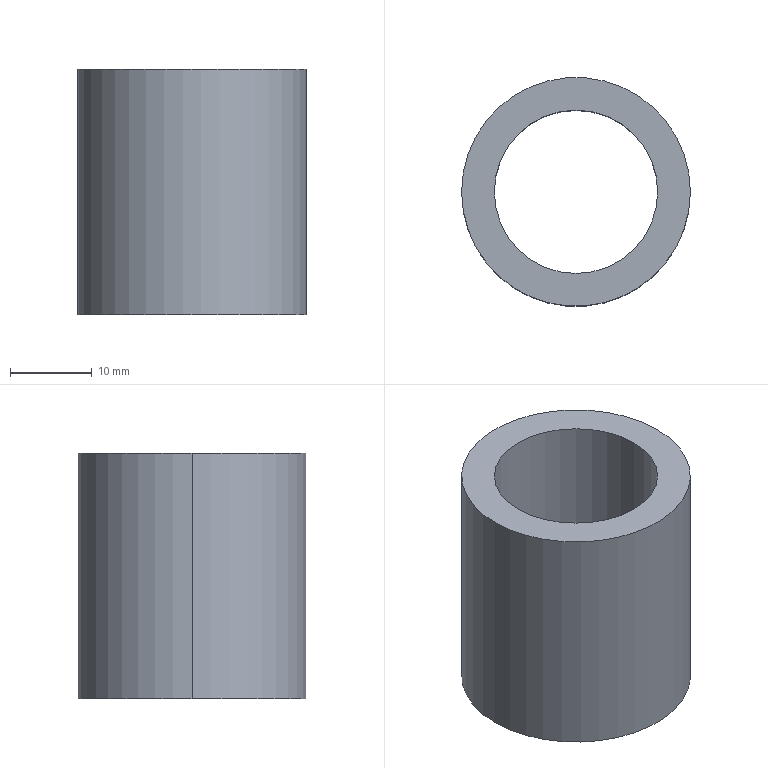Component | SolidWorks | GraphiteCopperSleeve2--1 | 1 solid | 6 faces | box 28 x 28 x 30 mm | volume 9048 mm3 | cylinder 4 | plane 2 | commonest cylinder face diameters 20 x2 28 x2
build123d program:
from build123d import *

# Parameters (mm, degrees)
SKETCH1_R           = 14
SKETCH1_R_2         = 10
BOSS_EXTRUDE1_DEPTH = 30


with BuildPart() as part:
    # Sketch1 → Boss-Extrude1 (new body)
    with BuildSketch(Plane.XY):
        Circle(SKETCH1_R)
        Circle(SKETCH1_R_2, mode=Mode.SUBTRACT)
    extrude(amount=BOSS_EXTRUDE1_DEPTH)


solid = part.part

# Placed as in the assembly
solid = solid.moved(Location((-372.766, -43.543, 885), (0, 0, 0)))
STEP:
#1=CARTESIAN_POINT('',(-15.07,-1.714,36.024));
#2=VERTEX_POINT('',#1);
#3=CARTESIAN_POINT('',(-14.282,-1.714,36.024));
#4=VERTEX_POINT('',#3);
#5=CARTESIAN_POINT('',(-14.676,-1.714,36.024));
#6=DIRECTION('',(0.,-0.,1.));
#7=DIRECTION('',(1.,0.,0.));
#8=AXIS2_PLACEMENT_3D('',#5,#6,#7);
#9=CIRCLE('',#8,0.3937);
#10=EDGE_CURVE('',#2,#4,#9,.T.);
#11=ORIENTED_EDGE('',*,*,#10,.T.);
#12=CARTESIAN_POINT('',(-14.282,-1.714,34.843));
#13=VERTEX_POINT('',#12);
#14=CARTESIAN_POINT('',(-14.282,-1.714,36.024));
#15=DIRECTION('',(-0.,0.,-1.));
#16=VECTOR('',#15,39.37);
#17=LINE('',#14,#16);
#18=EDGE_CURVE('',#4,#13,#17,.T.);
#19=ORIENTED_EDGE('',*,*,#18,.T.);
#20=CARTESIAN_POINT('',(-15.07,-1.714,34.843));
#21=VERTEX_POINT('',#20);
#22=CARTESIAN_POINT('',(-14.676,-1.714,34.843));
#23=DIRECTION('',(0.,-0.,1.));
#24=DIRECTION('',(1.,0.,0.));
#25=AXIS2_PLACEMENT_3D('',#22,#23,#24);
#26=CIRCLE('',#25,0.3937);
#27=EDGE_CURVE('',#21,#13,#26,.T.);
#28=ORIENTED_EDGE('',*,*,#27,.F.);
#29=CARTESIAN_POINT('',(-15.07,-1.714,36.024));
#30=DIRECTION('',(-0.,0.,-1.));
#31=VECTOR('',#30,39.37);
#32=LINE('',#29,#31);
#33=EDGE_CURVE('',#2,#21,#32,.T.);
#34=ORIENTED_EDGE('',*,*,#33,.F.);
#35=EDGE_LOOP('',(#11,#19,#28,#34));
#36=FACE_OUTER_BOUND('',#35,.T.);
#37=CARTESIAN_POINT('',(-14.676,-1.714,36.024));
#38=DIRECTION('',(-0.,0.,-1.));
#39=DIRECTION('',(-1.,-0.,0.));
#40=AXIS2_PLACEMENT_3D('',#37,#38,#39);
#41=CYLINDRICAL_SURFACE('',#40,0.3937);
#42=ADVANCED_FACE('',(#36),#41,.F.);
#43=CARTESIAN_POINT('',(-14.125,-1.714,36.024));
#44=VERTEX_POINT('',#43);
#45=CARTESIAN_POINT('',(-15.227,-1.714,36.024));
#46=VERTEX_POINT('',#45);
#47=CARTESIAN_POINT('',(-14.676,-1.714,36.024));
#48=DIRECTION('',(0.,-0.,1.));
#49=DIRECTION('',(1.,0.,0.));
#50=AXIS2_PLACEMENT_3D('',#47,#48,#49);
#51=CIRCLE('',#50,0.5512);
#52=EDGE_CURVE('',#44,#46,#51,.T.);
#53=ORIENTED_EDGE('',*,*,#52,.F.);
#54=CARTESIAN_POINT('',(-14.125,-1.714,34.843));
#55=VERTEX_POINT('',#54);
#56=CARTESIAN_POINT('',(-14.125,-1.714,36.024));
#57=DIRECTION('',(-0.,0.,-1.));
#58=VECTOR('',#57,39.37);
#59=LINE('',#56,#58);
#60=EDGE_CURVE('',#44,#55,#59,.T.);
#61=ORIENTED_EDGE('',*,*,#60,.T.);
#62=CARTESIAN_POINT('',(-15.227,-1.714,34.843));
#63=VERTEX_POINT('',#62);
#64=CARTESIAN_POINT('',(-14.676,-1.714,34.843));
#65=DIRECTION('',(0.,-0.,1.));
#66=DIRECTION('',(1.,0.,0.));
#67=AXIS2_PLACEMENT_3D('',#64,#65,#66);
#68=CIRCLE('',#67,0.5512);
#69=EDGE_CURVE('',#55,#63,#68,.T.);
#70=ORIENTED_EDGE('',*,*,#69,.T.);
#71=CARTESIAN_POINT('',(-15.227,-1.714,36.024));
#72=DIRECTION('',(-0.,0.,-1.));
#73=VECTOR('',#72,39.37);
#74=LINE('',#71,#73);
#75=EDGE_CURVE('',#46,#63,#74,.T.);
#76=ORIENTED_EDGE('',*,*,#75,.F.);
#77=EDGE_LOOP('',(#53,#61,#70,#76));
#78=FACE_OUTER_BOUND('',#77,.T.);
#79=CARTESIAN_POINT('',(-14.676,-1.714,36.024));
#80=DIRECTION('',(-0.,0.,-1.));
#81=DIRECTION('',(-1.,-0.,0.));
#82=AXIS2_PLACEMENT_3D('',#79,#80,#81);
#83=CYLINDRICAL_SURFACE('',#82,0.5512);
#84=ADVANCED_FACE('',(#78),#83,.T.);
#85=CARTESIAN_POINT('',(-14.676,-1.714,36.024));
#86=DIRECTION('',(0.,-0.,1.));
#87=DIRECTION('',(1.,0.,0.));
#88=AXIS2_PLACEMENT_3D('',#85,#86,#87);
#89=CIRCLE('',#88,0.5512);
#90=EDGE_CURVE('',#46,#44,#89,.T.);
#91=ORIENTED_EDGE('',*,*,#90,.T.);
#92=ORIENTED_EDGE('',*,*,#52,.T.);
#93=EDGE_LOOP('',(#91,#92));
#94=FACE_OUTER_BOUND('',#93,.T.);
#95=ORIENTED_EDGE('',*,*,#10,.F.);
#96=CARTESIAN_POINT('',(-14.676,-1.714,36.024));
#97=DIRECTION('',(0.,-0.,1.));
#98=DIRECTION('',(1.,0.,0.));
#99=AXIS2_PLACEMENT_3D('',#96,#97,#98);
#100=CIRCLE('',#99,0.3937);
#101=EDGE_CURVE('',#4,#2,#100,.T.);
#102=ORIENTED_EDGE('',*,*,#101,.F.);
#103=EDGE_LOOP('',(#95,#102));
#104=FACE_BOUND('',#103,.T.);
#105=CARTESIAN_POINT('',(-14.676,-1.714,36.024));
#106=DIRECTION('',(0.,-0.,1.));
#107=DIRECTION('',(1.,0.,-0.));
#108=AXIS2_PLACEMENT_3D('',#105,#106,#107);
#109=PLANE('',#108);
#110=ADVANCED_FACE('',(#94,#104),#109,.T.);
#111=CARTESIAN_POINT('',(-14.676,-1.714,34.843));
#112=DIRECTION('',(0.,-0.,1.));
#113=DIRECTION('',(1.,0.,0.));
#114=AXIS2_PLACEMENT_3D('',#111,#112,#113);
#115=CIRCLE('',#114,0.5512);
#116=EDGE_CURVE('',#63,#55,#115,.T.);
#117=ORIENTED_EDGE('',*,*,#116,.F.);
#118=ORIENTED_EDGE('',*,*,#69,.F.);
#119=EDGE_LOOP('',(#117,#118));
#120=FACE_OUTER_BOUND('',#119,.T.);
#121=ORIENTED_EDGE('',*,*,#27,.T.);
#122=CARTESIAN_POINT('',(-14.676,-1.714,34.843));
#123=DIRECTION('',(0.,-0.,1.));
#124=DIRECTION('',(1.,0.,0.));
#125=AXIS2_PLACEMENT_3D('',#122,#123,#124);
#126=CIRCLE('',#125,0.3937);
#127=EDGE_CURVE('',#13,#21,#126,.T.);
#128=ORIENTED_EDGE('',*,*,#127,.T.);
#129=EDGE_LOOP('',(#121,#128));
#130=FACE_BOUND('',#129,.T.);
#131=CARTESIAN_POINT('',(-14.676,-1.714,34.843));
#132=DIRECTION('',(0.,-0.,1.));
#133=DIRECTION('',(1.,0.,-0.));
#134=AXIS2_PLACEMENT_3D('',#131,#132,#133);
#135=PLANE('',#134);
#136=ADVANCED_FACE('',(#120,#130),#135,.F.);
#137=ORIENTED_EDGE('',*,*,#60,.F.);
#138=ORIENTED_EDGE('',*,*,#90,.F.);
#139=ORIENTED_EDGE('',*,*,#75,.T.);
#140=ORIENTED_EDGE('',*,*,#116,.T.);
#141=EDGE_LOOP('',(#137,#138,#139,#140));
#142=FACE_OUTER_BOUND('',#141,.T.);
#143=CARTESIAN_POINT('',(-14.676,-1.714,36.024));
#144=DIRECTION('',(-0.,0.,-1.));
#145=DIRECTION('',(-1.,-0.,0.));
#146=AXIS2_PLACEMENT_3D('',#143,#144,#145);
#147=CYLINDRICAL_SURFACE('',#146,0.5512);
#148=ADVANCED_FACE('',(#142),#147,.T.);
#149=ORIENTED_EDGE('',*,*,#18,.F.);
#150=ORIENTED_EDGE('',*,*,#101,.T.);
#151=ORIENTED_EDGE('',*,*,#33,.T.);
#152=ORIENTED_EDGE('',*,*,#127,.F.);
#153=EDGE_LOOP('',(#149,#150,#151,#152));
#154=FACE_OUTER_BOUND('',#153,.T.);
#155=CARTESIAN_POINT('',(-14.676,-1.714,36.024));
#156=DIRECTION('',(-0.,0.,-1.));
#157=DIRECTION('',(-1.,-0.,0.));
#158=AXIS2_PLACEMENT_3D('',#155,#156,#157);
#159=CYLINDRICAL_SURFACE('',#158,0.3937);
#160=ADVANCED_FACE('',(#154),#159,.F.);
#161=CLOSED_SHELL('',(#42,#84,#110,#136,#148,#160));
#162=MANIFOLD_SOLID_BREP('',#161);
#163=CARTESIAN_POINT('',(0.,0.,0.));
#164=DIRECTION('',(0.,0.,1.));
#165=DIRECTION('',(1.,0.,0.));
#166=AXIS2_PLACEMENT_3D('',#163,#164,#165);
#167=(LENGTH_UNIT()NAMED_UNIT(*)SI_UNIT($,.METRE.));
#168=LENGTH_MEASURE_WITH_UNIT(LENGTH_MEASURE(0.0254),#167);
#169=DIMENSIONAL_EXPONENTS(1.,0.,0.,0.,0.,0.,0.);
#170=(CONVERSION_BASED_UNIT('',#168)LENGTH_UNIT()NAMED_UNIT(#169));
#171=UNCERTAINTY_MEASURE_WITH_UNIT(LENGTH_MEASURE(0.00001),#170,'','');
#172=(NAMED_UNIT(*)PLANE_ANGLE_UNIT()SI_UNIT($,.RADIAN.));
#173=(NAMED_UNIT(*)SI_UNIT($,.STERADIAN.)SOLID_ANGLE_UNIT());
#174=(GEOMETRIC_REPRESENTATION_CONTEXT(3)GLOBAL_UNCERTAINTY_ASSIGNED_CONTEXT((#171))GLOBAL_UNIT_ASSIGNED_CONTEXT((#170,#172,#173))REPRESENTATION_CONTEXT('',''));
#175=ADVANCED_BREP_SHAPE_REPRESENTATION('',(#162,#166),#174);
#176=COLOUR_RGB('',0.7922,0.8196,0.9333);
#177=FILL_AREA_STYLE_COLOUR('',#176);
#178=FILL_AREA_STYLE('',(#177));
#179=SURFACE_STYLE_FILL_AREA(#178);
#180=SURFACE_SIDE_STYLE('',(#179));
#181=SURFACE_STYLE_USAGE(.BOTH.,#180);
#182=PRESENTATION_STYLE_ASSIGNMENT((#181));
#183=STYLED_ITEM('',(#182),#162);
#184=PRESENTATION_LAYER_ASSIGNMENT('','',(#183));
#185=(LENGTH_UNIT()NAMED_UNIT(*)SI_UNIT($,.METRE.));
#186=LENGTH_MEASURE_WITH_UNIT(LENGTH_MEASURE(0.0254),#185);
#187=DIMENSIONAL_EXPONENTS(1.,0.,0.,0.,0.,0.,0.);
#188=(CONVERSION_BASED_UNIT('',#186)LENGTH_UNIT()NAMED_UNIT(#187));
#189=UNCERTAINTY_MEASURE_WITH_UNIT(LENGTH_MEASURE(0.00001),#188,'','');
#190=(NAMED_UNIT(*)PLANE_ANGLE_UNIT()SI_UNIT($,.RADIAN.));
#191=(NAMED_UNIT(*)SI_UNIT($,.STERADIAN.)SOLID_ANGLE_UNIT());
#192=(GEOMETRIC_REPRESENTATION_CONTEXT(3)GLOBAL_UNCERTAINTY_ASSIGNED_CONTEXT((#189))GLOBAL_UNIT_ASSIGNED_CONTEXT((#188,#190,#191))REPRESENTATION_CONTEXT('',''));
#193=MECHANICAL_DESIGN_GEOMETRIC_PRESENTATION_REPRESENTATION('',(#183),#192);